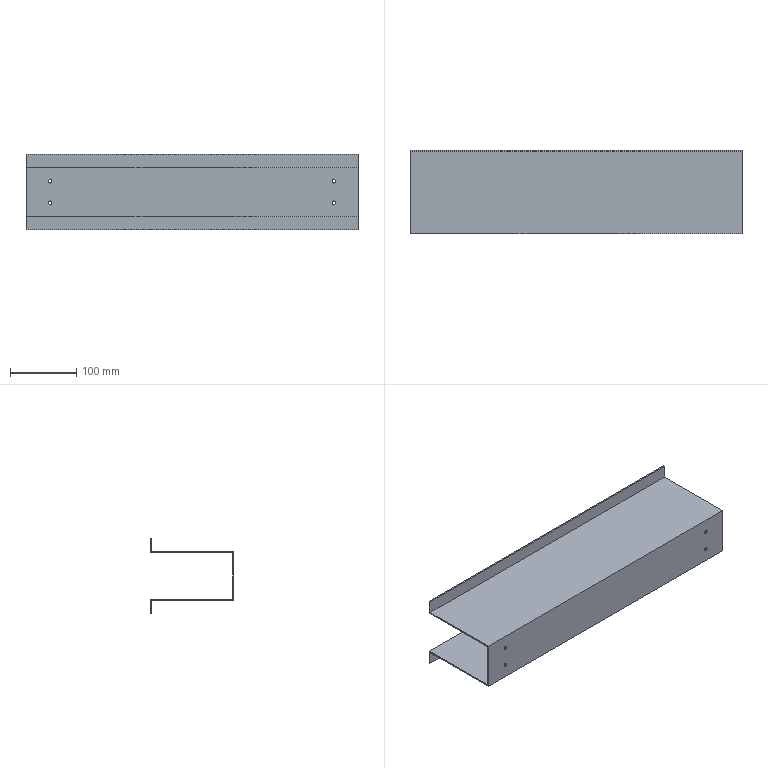Component | SolidWorks | LampHolder-1 | 1 solid | 22 faces | box 500 x 126 x 114 mm | volume 361830 mm3 | plane 14 | cylinder 8 | commonest cylinder face diameters 5.2 x8
build123d program:
from build123d import *

# Parameters (mm, degrees)
EXTRUDE_THIN1_DEPTH = 500
SKETCH2_R           = 2.6
CUT_EXTRUDE1_DEPTH  = 2


with BuildPart() as part:
    # Sketch1 → Extrude-Thin1 (new body)
    with BuildSketch(Plane.XY):
        Polygon((-52.485, -37.928), (-32.485, -37.928), (-32.485, 86.072), (41.515, 86.072), (41.515, -37.928), (61.515, -37.928), (61.515, -39.928), (39.515, -39.928), (39.515, 84.072), (-30.485, 84.072), (-30.485, -39.928), (-52.485, -39.928), align=None)
    extrude(amount=EXTRUDE_THIN1_DEPTH)

    # Sketch2 → Cut-Extrude1 (cut)
    with BuildSketch(Plane(origin=(0, 86.072, 0), x_dir=(1, 0, 0), z_dir=(0, 1, 0))):
        with Locations(Location((-11.485, -36.5, 0), (0, 0, 270))):
            Circle(SKETCH2_R)
        with Locations(Location((20.515, -36.5, 0), (0, 0, 270))):
            Circle(SKETCH2_R)
        with Locations(Location((-11.485, -463.5, 0), (0, 0, 270))):
            Circle(SKETCH2_R)
        with Locations(Location((20.515, -463.5, 0), (0, 0, 270))):
            Circle(SKETCH2_R)
    extrude(amount=-CUT_EXTRUDE1_DEPTH, mode=Mode.SUBTRACT)


solid = part.part

# Placed as in the assembly
solid = solid.moved(Location((-244.55, 457.638, -183.034), (180, 90, 0)))
STEP:
#1=CARTESIAN_POINT('',(8.518,14.707,-6.398));
#2=VERTEX_POINT('',#1);
#3=CARTESIAN_POINT('',(8.722,14.707,-6.398));
#4=VERTEX_POINT('',#3);
#5=CARTESIAN_POINT('',(8.62,14.707,-6.398));
#6=DIRECTION('',(0.,-1.,0.));
#7=DIRECTION('',(1.,0.,0.));
#8=AXIS2_PLACEMENT_3D('',#5,#6,#7);
#9=CIRCLE('',#8,0.1024);
#10=EDGE_CURVE('',#2,#4,#9,.T.);
#11=ORIENTED_EDGE('',*,*,#10,.F.);
#12=CARTESIAN_POINT('',(8.518,14.629,-6.398));
#13=VERTEX_POINT('',#12);
#14=CARTESIAN_POINT('',(8.518,14.707,-6.398));
#15=DIRECTION('',(0.,-1.,0.));
#16=VECTOR('',#15,39.37);
#17=LINE('',#14,#16);
#18=EDGE_CURVE('',#2,#13,#17,.T.);
#19=ORIENTED_EDGE('',*,*,#18,.T.);
#20=CARTESIAN_POINT('',(8.722,14.629,-6.398));
#21=VERTEX_POINT('',#20);
#22=CARTESIAN_POINT('',(8.62,14.629,-6.398));
#23=DIRECTION('',(0.,-1.,0.));
#24=DIRECTION('',(1.,0.,0.));
#25=AXIS2_PLACEMENT_3D('',#22,#23,#24);
#26=CIRCLE('',#25,0.1024);
#27=EDGE_CURVE('',#13,#21,#26,.T.);
#28=ORIENTED_EDGE('',*,*,#27,.T.);
#29=CARTESIAN_POINT('',(8.722,14.707,-6.398));
#30=DIRECTION('',(0.,-1.,0.));
#31=VECTOR('',#30,39.37);
#32=LINE('',#29,#31);
#33=EDGE_CURVE('',#4,#21,#32,.T.);
#34=ORIENTED_EDGE('',*,*,#33,.F.);
#35=EDGE_LOOP('',(#11,#19,#28,#34));
#36=FACE_OUTER_BOUND('',#35,.T.);
#37=CARTESIAN_POINT('',(8.62,14.707,-6.398));
#38=DIRECTION('',(0.,-1.,0.));
#39=DIRECTION('',(1.,0.,0.));
#40=AXIS2_PLACEMENT_3D('',#37,#38,#39);
#41=CYLINDRICAL_SURFACE('',#40,0.1024);
#42=ADVANCED_FACE('',(#36),#41,.F.);
#43=CARTESIAN_POINT('',(8.518,14.707,-7.658));
#44=VERTEX_POINT('',#43);
#45=CARTESIAN_POINT('',(8.722,14.707,-7.658));
#46=VERTEX_POINT('',#45);
#47=CARTESIAN_POINT('',(8.62,14.707,-7.658));
#48=DIRECTION('',(0.,-1.,0.));
#49=DIRECTION('',(1.,0.,0.));
#50=AXIS2_PLACEMENT_3D('',#47,#48,#49);
#51=CIRCLE('',#50,0.1024);
#52=EDGE_CURVE('',#44,#46,#51,.T.);
#53=ORIENTED_EDGE('',*,*,#52,.F.);
#54=CARTESIAN_POINT('',(8.518,14.629,-7.658));
#55=VERTEX_POINT('',#54);
#56=CARTESIAN_POINT('',(8.518,14.707,-7.658));
#57=DIRECTION('',(0.,-1.,0.));
#58=VECTOR('',#57,39.37);
#59=LINE('',#56,#58);
#60=EDGE_CURVE('',#44,#55,#59,.T.);
#61=ORIENTED_EDGE('',*,*,#60,.T.);
#62=CARTESIAN_POINT('',(8.722,14.629,-7.658));
#63=VERTEX_POINT('',#62);
#64=CARTESIAN_POINT('',(8.62,14.629,-7.658));
#65=DIRECTION('',(0.,-1.,0.));
#66=DIRECTION('',(1.,0.,0.));
#67=AXIS2_PLACEMENT_3D('',#64,#65,#66);
#68=CIRCLE('',#67,0.1024);
#69=EDGE_CURVE('',#55,#63,#68,.T.);
#70=ORIENTED_EDGE('',*,*,#69,.T.);
#71=CARTESIAN_POINT('',(8.722,14.707,-7.658));
#72=DIRECTION('',(0.,-1.,0.));
#73=VECTOR('',#72,39.37);
#74=LINE('',#71,#73);
#75=EDGE_CURVE('',#46,#63,#74,.T.);
#76=ORIENTED_EDGE('',*,*,#75,.F.);
#77=EDGE_LOOP('',(#53,#61,#70,#76));
#78=FACE_OUTER_BOUND('',#77,.T.);
#79=CARTESIAN_POINT('',(8.62,14.707,-7.658));
#80=DIRECTION('',(0.,-1.,0.));
#81=DIRECTION('',(1.,0.,0.));
#82=AXIS2_PLACEMENT_3D('',#79,#80,#81);
#83=CYLINDRICAL_SURFACE('',#82,0.1024);
#84=ADVANCED_FACE('',(#78),#83,.F.);
#85=CARTESIAN_POINT('',(-8.293,14.707,-6.398));
#86=VERTEX_POINT('',#85);
#87=CARTESIAN_POINT('',(-8.089,14.707,-6.398));
#88=VERTEX_POINT('',#87);
#89=CARTESIAN_POINT('',(-8.191,14.707,-6.398));
#90=DIRECTION('',(0.,-1.,0.));
#91=DIRECTION('',(1.,0.,0.));
#92=AXIS2_PLACEMENT_3D('',#89,#90,#91);
#93=CIRCLE('',#92,0.1024);
#94=EDGE_CURVE('',#86,#88,#93,.T.);
#95=ORIENTED_EDGE('',*,*,#94,.F.);
#96=CARTESIAN_POINT('',(-8.293,14.629,-6.398));
#97=VERTEX_POINT('',#96);
#98=CARTESIAN_POINT('',(-8.293,14.707,-6.398));
#99=DIRECTION('',(0.,-1.,0.));
#100=VECTOR('',#99,39.37);
#101=LINE('',#98,#100);
#102=EDGE_CURVE('',#86,#97,#101,.T.);
#103=ORIENTED_EDGE('',*,*,#102,.T.);
#104=CARTESIAN_POINT('',(-8.089,14.629,-6.398));
#105=VERTEX_POINT('',#104);
#106=CARTESIAN_POINT('',(-8.191,14.629,-6.398));
#107=DIRECTION('',(0.,-1.,0.));
#108=DIRECTION('',(1.,0.,0.));
#109=AXIS2_PLACEMENT_3D('',#106,#107,#108);
#110=CIRCLE('',#109,0.1024);
#111=EDGE_CURVE('',#97,#105,#110,.T.);
#112=ORIENTED_EDGE('',*,*,#111,.T.);
#113=CARTESIAN_POINT('',(-8.089,14.707,-6.398));
#114=DIRECTION('',(0.,-1.,0.));
#115=VECTOR('',#114,39.37);
#116=LINE('',#113,#115);
#117=EDGE_CURVE('',#88,#105,#116,.T.);
#118=ORIENTED_EDGE('',*,*,#117,.F.);
#119=EDGE_LOOP('',(#95,#103,#112,#118));
#120=FACE_OUTER_BOUND('',#119,.T.);
#121=CARTESIAN_POINT('',(-8.191,14.707,-6.398));
#122=DIRECTION('',(0.,-1.,0.));
#123=DIRECTION('',(1.,0.,0.));
#124=AXIS2_PLACEMENT_3D('',#121,#122,#123);
#125=CYLINDRICAL_SURFACE('',#124,0.1024);
#126=ADVANCED_FACE('',(#120),#125,.F.);
#127=CARTESIAN_POINT('',(-8.293,14.707,-7.658));
#128=VERTEX_POINT('',#127);
#129=CARTESIAN_POINT('',(-8.089,14.707,-7.658));
#130=VERTEX_POINT('',#129);
#131=CARTESIAN_POINT('',(-8.191,14.707,-7.658));
#132=DIRECTION('',(0.,-1.,0.));
#133=DIRECTION('',(1.,0.,0.));
#134=AXIS2_PLACEMENT_3D('',#131,#132,#133);
#135=CIRCLE('',#134,0.1024);
#136=EDGE_CURVE('',#128,#130,#135,.T.);
#137=ORIENTED_EDGE('',*,*,#136,.F.);
#138=CARTESIAN_POINT('',(-8.293,14.629,-7.658));
#139=VERTEX_POINT('',#138);
#140=CARTESIAN_POINT('',(-8.293,14.707,-7.658));
#141=DIRECTION('',(0.,-1.,0.));
#142=VECTOR('',#141,39.37);
#143=LINE('',#140,#142);
#144=EDGE_CURVE('',#128,#139,#143,.T.);
#145=ORIENTED_EDGE('',*,*,#144,.T.);
#146=CARTESIAN_POINT('',(-8.089,14.629,-7.658));
#147=VERTEX_POINT('',#146);
#148=CARTESIAN_POINT('',(-8.191,14.629,-7.658));
#149=DIRECTION('',(0.,-1.,0.));
#150=DIRECTION('',(1.,0.,0.));
#151=AXIS2_PLACEMENT_3D('',#148,#149,#150);
#152=CIRCLE('',#151,0.1024);
#153=EDGE_CURVE('',#139,#147,#152,.T.);
#154=ORIENTED_EDGE('',*,*,#153,.T.);
#155=CARTESIAN_POINT('',(-8.089,14.707,-7.658));
#156=DIRECTION('',(0.,-1.,0.));
#157=VECTOR('',#156,39.37);
#158=LINE('',#155,#157);
#159=EDGE_CURVE('',#130,#147,#158,.T.);
#160=ORIENTED_EDGE('',*,*,#159,.F.);
#161=EDGE_LOOP('',(#137,#145,#154,#160));
#162=FACE_OUTER_BOUND('',#161,.T.);
#163=CARTESIAN_POINT('',(-8.191,14.707,-7.658));
#164=DIRECTION('',(0.,-1.,0.));
#165=DIRECTION('',(1.,0.,0.));
#166=AXIS2_PLACEMENT_3D('',#163,#164,#165);
#167=CYLINDRICAL_SURFACE('',#166,0.1024);
#168=ADVANCED_FACE('',(#162),#167,.F.);
#169=CARTESIAN_POINT('',(-9.628,19.589,-5.65));
#170=VERTEX_POINT('',#169);
#171=CARTESIAN_POINT('',(-9.628,19.589,-4.784));
#172=VERTEX_POINT('',#171);
#173=CARTESIAN_POINT('',(-9.628,19.589,-5.572));
#174=DIRECTION('',(0.,0.,1.));
#175=VECTOR('',#174,39.37);
#176=LINE('',#173,#175);
#177=EDGE_CURVE('',#170,#172,#176,.T.);
#178=ORIENTED_EDGE('',*,*,#177,.T.);
#179=CARTESIAN_POINT('',(10.057,19.589,-4.784));
#180=VERTEX_POINT('',#179);
#181=CARTESIAN_POINT('',(10.057,19.589,-4.784));
#182=DIRECTION('',(-1.,-0.,0.));
#183=VECTOR('',#182,39.37);
#184=LINE('',#181,#183);
#185=EDGE_CURVE('',#180,#172,#184,.T.);
#186=ORIENTED_EDGE('',*,*,#185,.F.);
#187=CARTESIAN_POINT('',(10.057,19.589,-5.65));
#188=VERTEX_POINT('',#187);
#189=CARTESIAN_POINT('',(10.057,19.589,-5.572));
#190=DIRECTION('',(0.,0.,1.));
#191=VECTOR('',#190,39.37);
#192=LINE('',#189,#191);
#193=EDGE_CURVE('',#188,#180,#192,.T.);
#194=ORIENTED_EDGE('',*,*,#193,.F.);
#195=CARTESIAN_POINT('',(10.057,19.589,-5.65));
#196=DIRECTION('',(-1.,-0.,0.));
#197=VECTOR('',#196,39.37);
#198=LINE('',#195,#197);
#199=EDGE_CURVE('',#188,#170,#198,.T.);
#200=ORIENTED_EDGE('',*,*,#199,.T.);
#201=EDGE_LOOP('',(#178,#186,#194,#200));
#202=FACE_OUTER_BOUND('',#201,.T.);
#203=CARTESIAN_POINT('',(10.057,19.589,-5.572));
#204=DIRECTION('',(0.,-1.,0.));
#205=DIRECTION('',(1.,0.,-0.));
#206=AXIS2_PLACEMENT_3D('',#203,#204,#205);
#207=PLANE('',#206);
#208=ADVANCED_FACE('',(#202),#207,.F.);
#209=CARTESIAN_POINT('',(-9.628,19.51,-4.784));
#210=VERTEX_POINT('',#209);
#211=CARTESIAN_POINT('',(-9.628,19.51,-4.784));
#212=DIRECTION('',(-0.,1.,-0.));
#213=VECTOR('',#212,39.37);
#214=LINE('',#211,#213);
#215=EDGE_CURVE('',#210,#172,#214,.T.);
#216=ORIENTED_EDGE('',*,*,#215,.F.);
#217=CARTESIAN_POINT('',(10.057,19.51,-4.784));
#218=VERTEX_POINT('',#217);
#219=CARTESIAN_POINT('',(10.057,19.51,-4.784));
#220=DIRECTION('',(-1.,-0.,0.));
#221=VECTOR('',#220,39.37);
#222=LINE('',#219,#221);
#223=EDGE_CURVE('',#218,#210,#222,.T.);
#224=ORIENTED_EDGE('',*,*,#223,.F.);
#225=CARTESIAN_POINT('',(10.057,19.51,-4.784));
#226=DIRECTION('',(-0.,1.,-0.));
#227=VECTOR('',#226,39.37);
#228=LINE('',#225,#227);
#229=EDGE_CURVE('',#218,#180,#228,.T.);
#230=ORIENTED_EDGE('',*,*,#229,.T.);
#231=ORIENTED_EDGE('',*,*,#185,.T.);
#232=EDGE_LOOP('',(#216,#224,#230,#231));
#233=FACE_OUTER_BOUND('',#232,.T.);
#234=CARTESIAN_POINT('',(10.057,19.51,-4.784));
#235=DIRECTION('',(0.,0.,1.));
#236=DIRECTION('',(-1.,-0.,0.));
#237=AXIS2_PLACEMENT_3D('',#234,#235,#236);
#238=PLANE('',#237);
#239=ADVANCED_FACE('',(#233),#238,.T.);
#240=CARTESIAN_POINT('',(-9.628,19.51,-5.572));
#241=VERTEX_POINT('',#240);
#242=CARTESIAN_POINT('',(-9.628,19.51,-5.572));
#243=DIRECTION('',(0.,0.,1.));
#244=VECTOR('',#243,39.37);
#245=LINE('',#242,#244);
#246=EDGE_CURVE('',#241,#210,#245,.T.);
#247=ORIENTED_EDGE('',*,*,#246,.F.);
#248=CARTESIAN_POINT('',(10.057,19.51,-5.572));
#249=VERTEX_POINT('',#248);
#250=CARTESIAN_POINT('',(10.057,19.51,-5.572));
#251=DIRECTION('',(-1.,-0.,0.));
#252=VECTOR('',#251,39.37);
#253=LINE('',#250,#252);
#254=EDGE_CURVE('',#249,#241,#253,.T.);
#255=ORIENTED_EDGE('',*,*,#254,.F.);
#256=CARTESIAN_POINT('',(10.057,19.51,-5.572));
#257=DIRECTION('',(0.,0.,1.));
#258=VECTOR('',#257,39.37);
#259=LINE('',#256,#258);
#260=EDGE_CURVE('',#249,#218,#259,.T.);
#261=ORIENTED_EDGE('',*,*,#260,.T.);
#262=ORIENTED_EDGE('',*,*,#223,.T.);
#263=EDGE_LOOP('',(#247,#255,#261,#262));
#264=FACE_OUTER_BOUND('',#263,.T.);
#265=CARTESIAN_POINT('',(10.057,19.51,-5.572));
#266=DIRECTION('',(0.,-1.,0.));
#267=DIRECTION('',(1.,0.,-0.));
#268=AXIS2_PLACEMENT_3D('',#265,#266,#267);
#269=PLANE('',#268);
#270=ADVANCED_FACE('',(#264),#269,.T.);
#271=CARTESIAN_POINT('',(-9.628,14.629,-5.572));
#272=VERTEX_POINT('',#271);
#273=CARTESIAN_POINT('',(-9.628,14.629,-5.572));
#274=DIRECTION('',(-0.,1.,0.));
#275=VECTOR('',#274,39.37);
#276=LINE('',#273,#275);
#277=EDGE_CURVE('',#272,#241,#276,.T.);
#278=ORIENTED_EDGE('',*,*,#277,.F.);
#279=CARTESIAN_POINT('',(10.057,14.629,-5.572));
#280=VERTEX_POINT('',#279);
#281=CARTESIAN_POINT('',(10.057,14.629,-5.572));
#282=DIRECTION('',(-1.,-0.,0.));
#283=VECTOR('',#282,39.37);
#284=LINE('',#281,#283);
#285=EDGE_CURVE('',#280,#272,#284,.T.);
#286=ORIENTED_EDGE('',*,*,#285,.F.);
#287=CARTESIAN_POINT('',(10.057,14.629,-5.572));
#288=DIRECTION('',(-0.,1.,0.));
#289=VECTOR('',#288,39.37);
#290=LINE('',#287,#289);
#291=EDGE_CURVE('',#280,#249,#290,.T.);
#292=ORIENTED_EDGE('',*,*,#291,.T.);
#293=ORIENTED_EDGE('',*,*,#254,.T.);
#294=EDGE_LOOP('',(#278,#286,#292,#293));
#295=FACE_OUTER_BOUND('',#294,.T.);
#296=CARTESIAN_POINT('',(10.057,14.629,-5.572));
#297=DIRECTION('',(0.,-0.,1.));
#298=DIRECTION('',(0.,-1.,-0.));
#299=AXIS2_PLACEMENT_3D('',#296,#297,#298);
#300=PLANE('',#299);
#301=ADVANCED_FACE('',(#295),#300,.T.);
#302=CARTESIAN_POINT('',(8.62,14.629,-6.398));
#303=DIRECTION('',(0.,-1.,0.));
#304=DIRECTION('',(1.,0.,0.));
#305=AXIS2_PLACEMENT_3D('',#302,#303,#304);
#306=CIRCLE('',#305,0.1024);
#307=EDGE_CURVE('',#21,#13,#306,.T.);
#308=ORIENTED_EDGE('',*,*,#307,.F.);
#309=ORIENTED_EDGE('',*,*,#27,.F.);
#310=EDGE_LOOP('',(#308,#309));
#311=FACE_BOUND('',#310,.T.);
#312=CARTESIAN_POINT('',(8.62,14.629,-7.658));
#313=DIRECTION('',(0.,-1.,0.));
#314=DIRECTION('',(1.,0.,0.));
#315=AXIS2_PLACEMENT_3D('',#312,#313,#314);
#316=CIRCLE('',#315,0.1024);
#317=EDGE_CURVE('',#63,#55,#316,.T.);
#318=ORIENTED_EDGE('',*,*,#317,.F.);
#319=ORIENTED_EDGE('',*,*,#69,.F.);
#320=EDGE_LOOP('',(#318,#319));
#321=FACE_BOUND('',#320,.T.);
#322=CARTESIAN_POINT('',(-8.191,14.629,-6.398));
#323=DIRECTION('',(0.,-1.,0.));
#324=DIRECTION('',(1.,0.,0.));
#325=AXIS2_PLACEMENT_3D('',#322,#323,#324);
#326=CIRCLE('',#325,0.1024);
#327=EDGE_CURVE('',#105,#97,#326,.T.);
#328=ORIENTED_EDGE('',*,*,#327,.F.);
#329=ORIENTED_EDGE('',*,*,#111,.F.);
#330=EDGE_LOOP('',(#328,#329));
#331=FACE_BOUND('',#330,.T.);
#332=CARTESIAN_POINT('',(-8.191,14.629,-7.658));
#333=DIRECTION('',(0.,-1.,0.));
#334=DIRECTION('',(1.,0.,0.));
#335=AXIS2_PLACEMENT_3D('',#332,#333,#334);
#336=CIRCLE('',#335,0.1024);
#337=EDGE_CURVE('',#147,#139,#336,.T.);
#338=ORIENTED_EDGE('',*,*,#337,.F.);
#339=ORIENTED_EDGE('',*,*,#153,.F.);
#340=EDGE_LOOP('',(#338,#339));
#341=FACE_BOUND('',#340,.T.);
#342=CARTESIAN_POINT('',(-9.628,14.629,-8.485));
#343=VERTEX_POINT('',#342);
#344=CARTESIAN_POINT('',(-9.628,14.629,-8.485));
#345=DIRECTION('',(0.,0.,1.));
#346=VECTOR('',#345,39.37);
#347=LINE('',#344,#346);
#348=EDGE_CURVE('',#343,#272,#347,.T.);
#349=ORIENTED_EDGE('',*,*,#348,.F.);
#350=CARTESIAN_POINT('',(10.057,14.629,-8.485));
#351=VERTEX_POINT('',#350);
#352=CARTESIAN_POINT('',(10.057,14.629,-8.485));
#353=DIRECTION('',(-1.,-0.,0.));
#354=VECTOR('',#353,39.37);
#355=LINE('',#352,#354);
#356=EDGE_CURVE('',#351,#343,#355,.T.);
#357=ORIENTED_EDGE('',*,*,#356,.F.);
#358=CARTESIAN_POINT('',(10.057,14.629,-8.485));
#359=DIRECTION('',(0.,0.,1.));
#360=VECTOR('',#359,39.37);
#361=LINE('',#358,#360);
#362=EDGE_CURVE('',#351,#280,#361,.T.);
#363=ORIENTED_EDGE('',*,*,#362,.T.);
#364=ORIENTED_EDGE('',*,*,#285,.T.);
#365=EDGE_LOOP('',(#349,#357,#363,#364));
#366=FACE_OUTER_BOUND('',#365,.T.);
#367=CARTESIAN_POINT('',(10.057,14.629,-8.485));
#368=DIRECTION('',(0.,-1.,0.));
#369=DIRECTION('',(1.,0.,-0.));
#370=AXIS2_PLACEMENT_3D('',#367,#368,#369);
#371=PLANE('',#370);
#372=ADVANCED_FACE('',(#311,#321,#331,#341,#366),#371,.T.);
#373=CARTESIAN_POINT('',(-9.628,19.51,-8.485));
#374=VERTEX_POINT('',#373);
#375=CARTESIAN_POINT('',(-9.628,19.51,-8.485));
#376=DIRECTION('',(0.,-1.,-0.));
#377=VECTOR('',#376,39.37);
#378=LINE('',#375,#377);
#379=EDGE_CURVE('',#374,#343,#378,.T.);
#380=ORIENTED_EDGE('',*,*,#379,.F.);
#381=CARTESIAN_POINT('',(10.057,19.51,-8.485));
#382=VERTEX_POINT('',#381);
#383=CARTESIAN_POINT('',(10.057,19.51,-8.485));
#384=DIRECTION('',(-1.,-0.,0.));
#385=VECTOR('',#384,39.37);
#386=LINE('',#383,#385);
#387=EDGE_CURVE('',#382,#374,#386,.T.);
#388=ORIENTED_EDGE('',*,*,#387,.F.);
#389=CARTESIAN_POINT('',(10.057,19.51,-8.485));
#390=DIRECTION('',(0.,-1.,-0.));
#391=VECTOR('',#390,39.37);
#392=LINE('',#389,#391);
#393=EDGE_CURVE('',#382,#351,#392,.T.);
#394=ORIENTED_EDGE('',*,*,#393,.T.);
#395=ORIENTED_EDGE('',*,*,#356,.T.);
#396=EDGE_LOOP('',(#380,#388,#394,#395));
#397=FACE_OUTER_BOUND('',#396,.T.);
#398=CARTESIAN_POINT('',(10.057,19.51,-8.485));
#399=DIRECTION('',(-0.,0.,-1.));
#400=DIRECTION('',(-0.,1.,0.));
#401=AXIS2_PLACEMENT_3D('',#398,#399,#400);
#402=PLANE('',#401);
#403=ADVANCED_FACE('',(#397),#402,.T.);
#404=CARTESIAN_POINT('',(-9.628,19.51,-9.272));
#405=VERTEX_POINT('',#404);
#406=CARTESIAN_POINT('',(-9.628,19.51,-9.272));
#407=DIRECTION('',(0.,0.,1.));
#408=VECTOR('',#407,39.37);
#409=LINE('',#406,#408);
#410=EDGE_CURVE('',#405,#374,#409,.T.);
#411=ORIENTED_EDGE('',*,*,#410,.F.);
#412=CARTESIAN_POINT('',(10.057,19.51,-9.272));
#413=VERTEX_POINT('',#412);
#414=CARTESIAN_POINT('',(10.057,19.51,-9.272));
#415=DIRECTION('',(-1.,-0.,0.));
#416=VECTOR('',#415,39.37);
#417=LINE('',#414,#416);
#418=EDGE_CURVE('',#413,#405,#417,.T.);
#419=ORIENTED_EDGE('',*,*,#418,.F.);
#420=CARTESIAN_POINT('',(10.057,19.51,-9.272));
#421=DIRECTION('',(0.,0.,1.));
#422=VECTOR('',#421,39.37);
#423=LINE('',#420,#422);
#424=EDGE_CURVE('',#413,#382,#423,.T.);
#425=ORIENTED_EDGE('',*,*,#424,.T.);
#426=ORIENTED_EDGE('',*,*,#387,.T.);
#427=EDGE_LOOP('',(#411,#419,#425,#426));
#428=FACE_OUTER_BOUND('',#427,.T.);
#429=CARTESIAN_POINT('',(10.057,19.51,-9.272));
#430=DIRECTION('',(0.,-1.,0.));
#431=DIRECTION('',(1.,0.,-0.));
#432=AXIS2_PLACEMENT_3D('',#429,#430,#431);
#433=PLANE('',#432);
#434=ADVANCED_FACE('',(#428),#433,.T.);
#435=CARTESIAN_POINT('',(-9.628,19.589,-9.272));
#436=VERTEX_POINT('',#435);
#437=CARTESIAN_POINT('',(-9.628,19.589,-9.272));
#438=DIRECTION('',(0.,-1.,0.));
#439=VECTOR('',#438,39.37);
#440=LINE('',#437,#439);
#441=EDGE_CURVE('',#436,#405,#440,.T.);
#442=ORIENTED_EDGE('',*,*,#441,.F.);
#443=CARTESIAN_POINT('',(10.057,19.589,-9.272));
#444=VERTEX_POINT('',#443);
#445=CARTESIAN_POINT('',(10.057,19.589,-9.272));
#446=DIRECTION('',(-1.,-0.,0.));
#447=VECTOR('',#446,39.37);
#448=LINE('',#445,#447);
#449=EDGE_CURVE('',#444,#436,#448,.T.);
#450=ORIENTED_EDGE('',*,*,#449,.F.);
#451=CARTESIAN_POINT('',(10.057,19.589,-9.272));
#452=DIRECTION('',(0.,-1.,0.));
#453=VECTOR('',#452,39.37);
#454=LINE('',#451,#453);
#455=EDGE_CURVE('',#444,#413,#454,.T.);
#456=ORIENTED_EDGE('',*,*,#455,.T.);
#457=ORIENTED_EDGE('',*,*,#418,.T.);
#458=EDGE_LOOP('',(#442,#450,#456,#457));
#459=FACE_OUTER_BOUND('',#458,.T.);
#460=CARTESIAN_POINT('',(10.057,19.589,-9.272));
#461=DIRECTION('',(-0.,-0.,-1.));
#462=DIRECTION('',(1.,0.,-0.));
#463=AXIS2_PLACEMENT_3D('',#460,#461,#462);
#464=PLANE('',#463);
#465=ADVANCED_FACE('',(#459),#464,.T.);
#466=CARTESIAN_POINT('',(-9.628,19.589,-8.406));
#467=VERTEX_POINT('',#466);
#468=CARTESIAN_POINT('',(-9.628,19.589,-9.272));
#469=DIRECTION('',(0.,0.,1.));
#470=VECTOR('',#469,39.37);
#471=LINE('',#468,#470);
#472=EDGE_CURVE('',#436,#467,#471,.T.);
#473=ORIENTED_EDGE('',*,*,#472,.T.);
#474=CARTESIAN_POINT('',(10.057,19.589,-8.406));
#475=VERTEX_POINT('',#474);
#476=CARTESIAN_POINT('',(10.057,19.589,-8.406));
#477=DIRECTION('',(-1.,-0.,0.));
#478=VECTOR('',#477,39.37);
#479=LINE('',#476,#478);
#480=EDGE_CURVE('',#475,#467,#479,.T.);
#481=ORIENTED_EDGE('',*,*,#480,.F.);
#482=CARTESIAN_POINT('',(10.057,19.589,-9.272));
#483=DIRECTION('',(0.,0.,1.));
#484=VECTOR('',#483,39.37);
#485=LINE('',#482,#484);
#486=EDGE_CURVE('',#444,#475,#485,.T.);
#487=ORIENTED_EDGE('',*,*,#486,.F.);
#488=ORIENTED_EDGE('',*,*,#449,.T.);
#489=EDGE_LOOP('',(#473,#481,#487,#488));
#490=FACE_OUTER_BOUND('',#489,.T.);
#491=CARTESIAN_POINT('',(10.057,19.589,-9.272));
#492=DIRECTION('',(0.,-1.,0.));
#493=DIRECTION('',(1.,0.,-0.));
#494=AXIS2_PLACEMENT_3D('',#491,#492,#493);
#495=PLANE('',#494);
#496=ADVANCED_FACE('',(#490),#495,.F.);
#497=CARTESIAN_POINT('',(-9.628,14.707,-8.406));
#498=VERTEX_POINT('',#497);
#499=CARTESIAN_POINT('',(-9.628,19.51,-8.406));
#500=DIRECTION('',(0.,-1.,-0.));
#501=VECTOR('',#500,39.37);
#502=LINE('',#499,#501);
#503=EDGE_CURVE('',#467,#498,#502,.T.);
#504=ORIENTED_EDGE('',*,*,#503,.T.);
#505=CARTESIAN_POINT('',(10.057,14.707,-8.406));
#506=VERTEX_POINT('',#505);
#507=CARTESIAN_POINT('',(10.057,14.707,-8.406));
#508=DIRECTION('',(-1.,-0.,0.));
#509=VECTOR('',#508,39.37);
#510=LINE('',#507,#509);
#511=EDGE_CURVE('',#506,#498,#510,.T.);
#512=ORIENTED_EDGE('',*,*,#511,.F.);
#513=CARTESIAN_POINT('',(10.057,19.51,-8.406));
#514=DIRECTION('',(0.,-1.,-0.));
#515=VECTOR('',#514,39.37);
#516=LINE('',#513,#515);
#517=EDGE_CURVE('',#475,#506,#516,.T.);
#518=ORIENTED_EDGE('',*,*,#517,.F.);
#519=ORIENTED_EDGE('',*,*,#480,.T.);
#520=EDGE_LOOP('',(#504,#512,#518,#519));
#521=FACE_OUTER_BOUND('',#520,.T.);
#522=CARTESIAN_POINT('',(10.057,19.51,-8.406));
#523=DIRECTION('',(-0.,0.,-1.));
#524=DIRECTION('',(-0.,1.,0.));
#525=AXIS2_PLACEMENT_3D('',#522,#523,#524);
#526=PLANE('',#525);
#527=ADVANCED_FACE('',(#521),#526,.F.);
#528=CARTESIAN_POINT('',(8.62,14.707,-6.398));
#529=DIRECTION('',(0.,-1.,0.));
#530=DIRECTION('',(1.,0.,0.));
#531=AXIS2_PLACEMENT_3D('',#528,#529,#530);
#532=CIRCLE('',#531,0.1024);
#533=EDGE_CURVE('',#4,#2,#532,.T.);
#534=ORIENTED_EDGE('',*,*,#533,.T.);
#535=ORIENTED_EDGE('',*,*,#10,.T.);
#536=EDGE_LOOP('',(#534,#535));
#537=FACE_BOUND('',#536,.T.);
#538=CARTESIAN_POINT('',(8.62,14.707,-7.658));
#539=DIRECTION('',(0.,-1.,0.));
#540=DIRECTION('',(1.,0.,0.));
#541=AXIS2_PLACEMENT_3D('',#538,#539,#540);
#542=CIRCLE('',#541,0.1024);
#543=EDGE_CURVE('',#46,#44,#542,.T.);
#544=ORIENTED_EDGE('',*,*,#543,.T.);
#545=ORIENTED_EDGE('',*,*,#52,.T.);
#546=EDGE_LOOP('',(#544,#545));
#547=FACE_BOUND('',#546,.T.);
#548=CARTESIAN_POINT('',(-8.191,14.707,-6.398));
#549=DIRECTION('',(0.,-1.,0.));
#550=DIRECTION('',(1.,0.,0.));
#551=AXIS2_PLACEMENT_3D('',#548,#549,#550);
#552=CIRCLE('',#551,0.1024);
#553=EDGE_CURVE('',#88,#86,#552,.T.);
#554=ORIENTED_EDGE('',*,*,#553,.T.);
#555=ORIENTED_EDGE('',*,*,#94,.T.);
#556=EDGE_LOOP('',(#554,#555));
#557=FACE_BOUND('',#556,.T.);
#558=CARTESIAN_POINT('',(-8.191,14.707,-7.658));
#559=DIRECTION('',(0.,-1.,0.));
#560=DIRECTION('',(1.,0.,0.));
#561=AXIS2_PLACEMENT_3D('',#558,#559,#560);
#562=CIRCLE('',#561,0.1024);
#563=EDGE_CURVE('',#130,#128,#562,.T.);
#564=ORIENTED_EDGE('',*,*,#563,.T.);
#565=ORIENTED_EDGE('',*,*,#136,.T.);
#566=EDGE_LOOP('',(#564,#565));
#567=FACE_BOUND('',#566,.T.);
#568=CARTESIAN_POINT('',(-9.628,14.707,-5.65));
#569=VERTEX_POINT('',#568);
#570=CARTESIAN_POINT('',(-9.628,14.707,-8.485));
#571=DIRECTION('',(0.,0.,1.));
#572=VECTOR('',#571,39.37);
#573=LINE('',#570,#572);
#574=EDGE_CURVE('',#498,#569,#573,.T.);
#575=ORIENTED_EDGE('',*,*,#574,.T.);
#576=CARTESIAN_POINT('',(10.057,14.707,-5.65));
#577=VERTEX_POINT('',#576);
#578=CARTESIAN_POINT('',(10.057,14.707,-5.65));
#579=DIRECTION('',(-1.,-0.,0.));
#580=VECTOR('',#579,39.37);
#581=LINE('',#578,#580);
#582=EDGE_CURVE('',#577,#569,#581,.T.);
#583=ORIENTED_EDGE('',*,*,#582,.F.);
#584=CARTESIAN_POINT('',(10.057,14.707,-8.485));
#585=DIRECTION('',(0.,0.,1.));
#586=VECTOR('',#585,39.37);
#587=LINE('',#584,#586);
#588=EDGE_CURVE('',#506,#577,#587,.T.);
#589=ORIENTED_EDGE('',*,*,#588,.F.);
#590=ORIENTED_EDGE('',*,*,#511,.T.);
#591=EDGE_LOOP('',(#575,#583,#589,#590));
#592=FACE_OUTER_BOUND('',#591,.T.);
#593=CARTESIAN_POINT('',(10.057,14.707,-8.485));
#594=DIRECTION('',(0.,-1.,0.));
#595=DIRECTION('',(1.,0.,-0.));
#596=AXIS2_PLACEMENT_3D('',#593,#594,#595);
#597=PLANE('',#596);
#598=ADVANCED_FACE('',(#537,#547,#557,#567,#592),#597,.F.);
#599=CARTESIAN_POINT('',(-9.628,14.629,-5.65));
#600=DIRECTION('',(-0.,1.,0.));
#601=VECTOR('',#600,39.37);
#602=LINE('',#599,#601);
#603=EDGE_CURVE('',#569,#170,#602,.T.);
#604=ORIENTED_EDGE('',*,*,#603,.T.);
#605=ORIENTED_EDGE('',*,*,#199,.F.);
#606=CARTESIAN_POINT('',(10.057,14.629,-5.65));
#607=DIRECTION('',(-0.,1.,0.));
#608=VECTOR('',#607,39.37);
#609=LINE('',#606,#608);
#610=EDGE_CURVE('',#577,#188,#609,.T.);
#611=ORIENTED_EDGE('',*,*,#610,.F.);
#612=ORIENTED_EDGE('',*,*,#582,.T.);
#613=EDGE_LOOP('',(#604,#605,#611,#612));
#614=FACE_OUTER_BOUND('',#613,.T.);
#615=CARTESIAN_POINT('',(10.057,14.629,-5.65));
#616=DIRECTION('',(0.,-0.,1.));
#617=DIRECTION('',(0.,-1.,-0.));
#618=AXIS2_PLACEMENT_3D('',#615,#616,#617);
#619=PLANE('',#618);
#620=ADVANCED_FACE('',(#614),#619,.F.);
#621=ORIENTED_EDGE('',*,*,#193,.T.);
#622=ORIENTED_EDGE('',*,*,#229,.F.);
#623=ORIENTED_EDGE('',*,*,#260,.F.);
#624=ORIENTED_EDGE('',*,*,#291,.F.);
#625=ORIENTED_EDGE('',*,*,#362,.F.);
#626=ORIENTED_EDGE('',*,*,#393,.F.);
#627=ORIENTED_EDGE('',*,*,#424,.F.);
#628=ORIENTED_EDGE('',*,*,#455,.F.);
#629=ORIENTED_EDGE('',*,*,#486,.T.);
#630=ORIENTED_EDGE('',*,*,#517,.T.);
#631=ORIENTED_EDGE('',*,*,#588,.T.);
#632=ORIENTED_EDGE('',*,*,#610,.T.);
#633=EDGE_LOOP('',(#621,#622,#623,#624,#625,#626,#627,#628,#629,#630,#631,#632));
#634=FACE_OUTER_BOUND('',#633,.T.);
#635=CARTESIAN_POINT('',(10.057,18.017,-7.206));
#636=DIRECTION('',(-1.,-0.,0.));
#637=DIRECTION('',(0.,0.,-1.));
#638=AXIS2_PLACEMENT_3D('',#635,#636,#637);
#639=PLANE('',#638);
#640=ADVANCED_FACE('',(#634),#639,.F.);
#641=ORIENTED_EDGE('',*,*,#177,.F.);
#642=ORIENTED_EDGE('',*,*,#603,.F.);
#643=ORIENTED_EDGE('',*,*,#574,.F.);
#644=ORIENTED_EDGE('',*,*,#503,.F.);
#645=ORIENTED_EDGE('',*,*,#472,.F.);
#646=ORIENTED_EDGE('',*,*,#441,.T.);
#647=ORIENTED_EDGE('',*,*,#410,.T.);
#648=ORIENTED_EDGE('',*,*,#379,.T.);
#649=ORIENTED_EDGE('',*,*,#348,.T.);
#650=ORIENTED_EDGE('',*,*,#277,.T.);
#651=ORIENTED_EDGE('',*,*,#246,.T.);
#652=ORIENTED_EDGE('',*,*,#215,.T.);
#653=EDGE_LOOP('',(#641,#642,#643,#644,#645,#646,#647,#648,#649,#650,#651,#652));
#654=FACE_OUTER_BOUND('',#653,.T.);
#655=CARTESIAN_POINT('',(-9.628,18.017,-7.206));
#656=DIRECTION('',(-1.,-0.,0.));
#657=DIRECTION('',(0.,0.,-1.));
#658=AXIS2_PLACEMENT_3D('',#655,#656,#657);
#659=PLANE('',#658);
#660=ADVANCED_FACE('',(#654),#659,.T.);
#661=ORIENTED_EDGE('',*,*,#144,.F.);
#662=ORIENTED_EDGE('',*,*,#563,.F.);
#663=ORIENTED_EDGE('',*,*,#159,.T.);
#664=ORIENTED_EDGE('',*,*,#337,.T.);
#665=EDGE_LOOP('',(#661,#662,#663,#664));
#666=FACE_OUTER_BOUND('',#665,.T.);
#667=CARTESIAN_POINT('',(-8.191,14.707,-7.658));
#668=DIRECTION('',(0.,-1.,0.));
#669=DIRECTION('',(1.,0.,0.));
#670=AXIS2_PLACEMENT_3D('',#667,#668,#669);
#671=CYLINDRICAL_SURFACE('',#670,0.1024);
#672=ADVANCED_FACE('',(#666),#671,.F.);
#673=ORIENTED_EDGE('',*,*,#102,.F.);
#674=ORIENTED_EDGE('',*,*,#553,.F.);
#675=ORIENTED_EDGE('',*,*,#117,.T.);
#676=ORIENTED_EDGE('',*,*,#327,.T.);
#677=EDGE_LOOP('',(#673,#674,#675,#676));
#678=FACE_OUTER_BOUND('',#677,.T.);
#679=CARTESIAN_POINT('',(-8.191,14.707,-6.398));
#680=DIRECTION('',(0.,-1.,0.));
#681=DIRECTION('',(1.,0.,0.));
#682=AXIS2_PLACEMENT_3D('',#679,#680,#681);
#683=CYLINDRICAL_SURFACE('',#682,0.1024);
#684=ADVANCED_FACE('',(#678),#683,.F.);
#685=ORIENTED_EDGE('',*,*,#60,.F.);
#686=ORIENTED_EDGE('',*,*,#543,.F.);
#687=ORIENTED_EDGE('',*,*,#75,.T.);
#688=ORIENTED_EDGE('',*,*,#317,.T.);
#689=EDGE_LOOP('',(#685,#686,#687,#688));
#690=FACE_OUTER_BOUND('',#689,.T.);
#691=CARTESIAN_POINT('',(8.62,14.707,-7.658));
#692=DIRECTION('',(0.,-1.,0.));
#693=DIRECTION('',(1.,0.,0.));
#694=AXIS2_PLACEMENT_3D('',#691,#692,#693);
#695=CYLINDRICAL_SURFACE('',#694,0.1024);
#696=ADVANCED_FACE('',(#690),#695,.F.);
#697=ORIENTED_EDGE('',*,*,#18,.F.);
#698=ORIENTED_EDGE('',*,*,#533,.F.);
#699=ORIENTED_EDGE('',*,*,#33,.T.);
#700=ORIENTED_EDGE('',*,*,#307,.T.);
#701=EDGE_LOOP('',(#697,#698,#699,#700));
#702=FACE_OUTER_BOUND('',#701,.T.);
#703=CARTESIAN_POINT('',(8.62,14.707,-6.398));
#704=DIRECTION('',(0.,-1.,0.));
#705=DIRECTION('',(1.,0.,0.));
#706=AXIS2_PLACEMENT_3D('',#703,#704,#705);
#707=CYLINDRICAL_SURFACE('',#706,0.1024);
#708=ADVANCED_FACE('',(#702),#707,.F.);
#709=CLOSED_SHELL('',(#42,#84,#126,#168,#208,#239,#270,#301,#372,#403,#434,#465,#496,#527,#598,#620,#640,#660,#672,#684,#696,#708));
#710=MANIFOLD_SOLID_BREP('',#709);
#711=CARTESIAN_POINT('',(0.,0.,0.));
#712=DIRECTION('',(0.,0.,1.));
#713=DIRECTION('',(1.,0.,0.));
#714=AXIS2_PLACEMENT_3D('',#711,#712,#713);
#715=(LENGTH_UNIT()NAMED_UNIT(*)SI_UNIT($,.METRE.));
#716=LENGTH_MEASURE_WITH_UNIT(LENGTH_MEASURE(0.0254),#715);
#717=DIMENSIONAL_EXPONENTS(1.,0.,0.,0.,0.,0.,0.);
#718=(CONVERSION_BASED_UNIT('',#716)LENGTH_UNIT()NAMED_UNIT(#717));
#719=UNCERTAINTY_MEASURE_WITH_UNIT(LENGTH_MEASURE(0.00001),#718,'','');
#720=(NAMED_UNIT(*)PLANE_ANGLE_UNIT()SI_UNIT($,.RADIAN.));
#721=(NAMED_UNIT(*)SI_UNIT($,.STERADIAN.)SOLID_ANGLE_UNIT());
#722=(GEOMETRIC_REPRESENTATION_CONTEXT(3)GLOBAL_UNCERTAINTY_ASSIGNED_CONTEXT((#719))GLOBAL_UNIT_ASSIGNED_CONTEXT((#718,#720,#721))REPRESENTATION_CONTEXT('',''));
#723=ADVANCED_BREP_SHAPE_REPRESENTATION('',(#710,#714),#722);
#724=COLOUR_RGB('',0.7922,0.8196,0.9333);
#725=FILL_AREA_STYLE_COLOUR('',#724);
#726=FILL_AREA_STYLE('',(#725));
#727=SURFACE_STYLE_FILL_AREA(#726);
#728=SURFACE_SIDE_STYLE('',(#727));
#729=SURFACE_STYLE_USAGE(.BOTH.,#728);
#730=PRESENTATION_STYLE_ASSIGNMENT((#729));
#731=STYLED_ITEM('',(#730),#710);
#732=PRESENTATION_LAYER_ASSIGNMENT('','',(#731));
#733=(LENGTH_UNIT()NAMED_UNIT(*)SI_UNIT($,.METRE.));
#734=LENGTH_MEASURE_WITH_UNIT(LENGTH_MEASURE(0.0254),#733);
#735=DIMENSIONAL_EXPONENTS(1.,0.,0.,0.,0.,0.,0.);
#736=(CONVERSION_BASED_UNIT('',#734)LENGTH_UNIT()NAMED_UNIT(#735));
#737=UNCERTAINTY_MEASURE_WITH_UNIT(LENGTH_MEASURE(0.00001),#736,'','');
#738=(NAMED_UNIT(*)PLANE_ANGLE_UNIT()SI_UNIT($,.RADIAN.));
#739=(NAMED_UNIT(*)SI_UNIT($,.STERADIAN.)SOLID_ANGLE_UNIT());
#740=(GEOMETRIC_REPRESENTATION_CONTEXT(3)GLOBAL_UNCERTAINTY_ASSIGNED_CONTEXT((#737))GLOBAL_UNIT_ASSIGNED_CONTEXT((#736,#738,#739))REPRESENTATION_CONTEXT('',''));
#741=MECHANICAL_DESIGN_GEOMETRIC_PRESENTATION_REPRESENTATION('',(#731),#740);